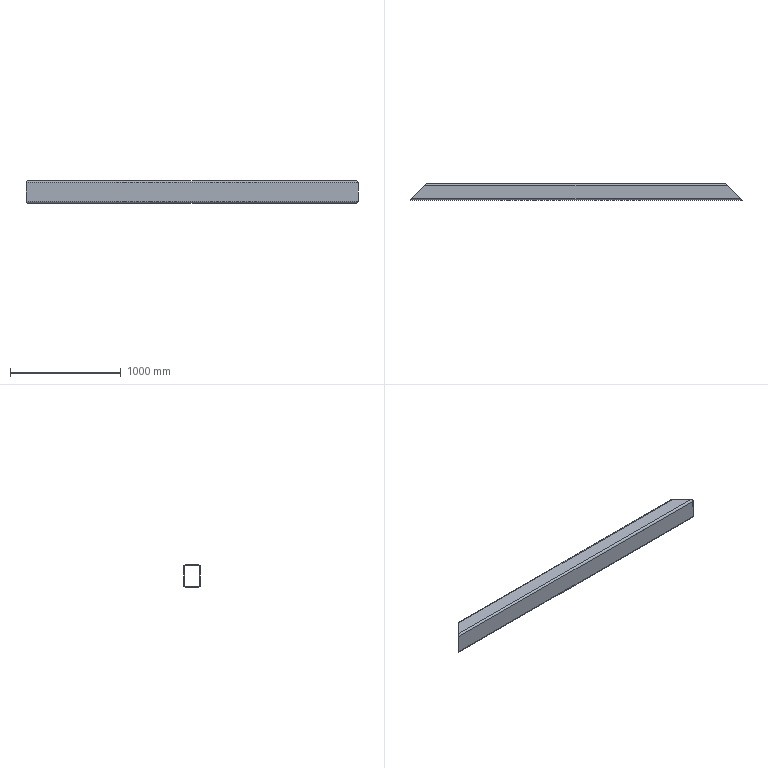Component | NX | AAAAAAAAAAAAAAAAAAAAAAAAAAAAAAAAAAAAAAAAAAAAAAAAAAAAAAAAAAA_13 | 1 solid | 18 faces | volume 14760680 mm3 | plane 10 | cylinder 8 | commonest cylinder face diameters 32 x4 16 x4